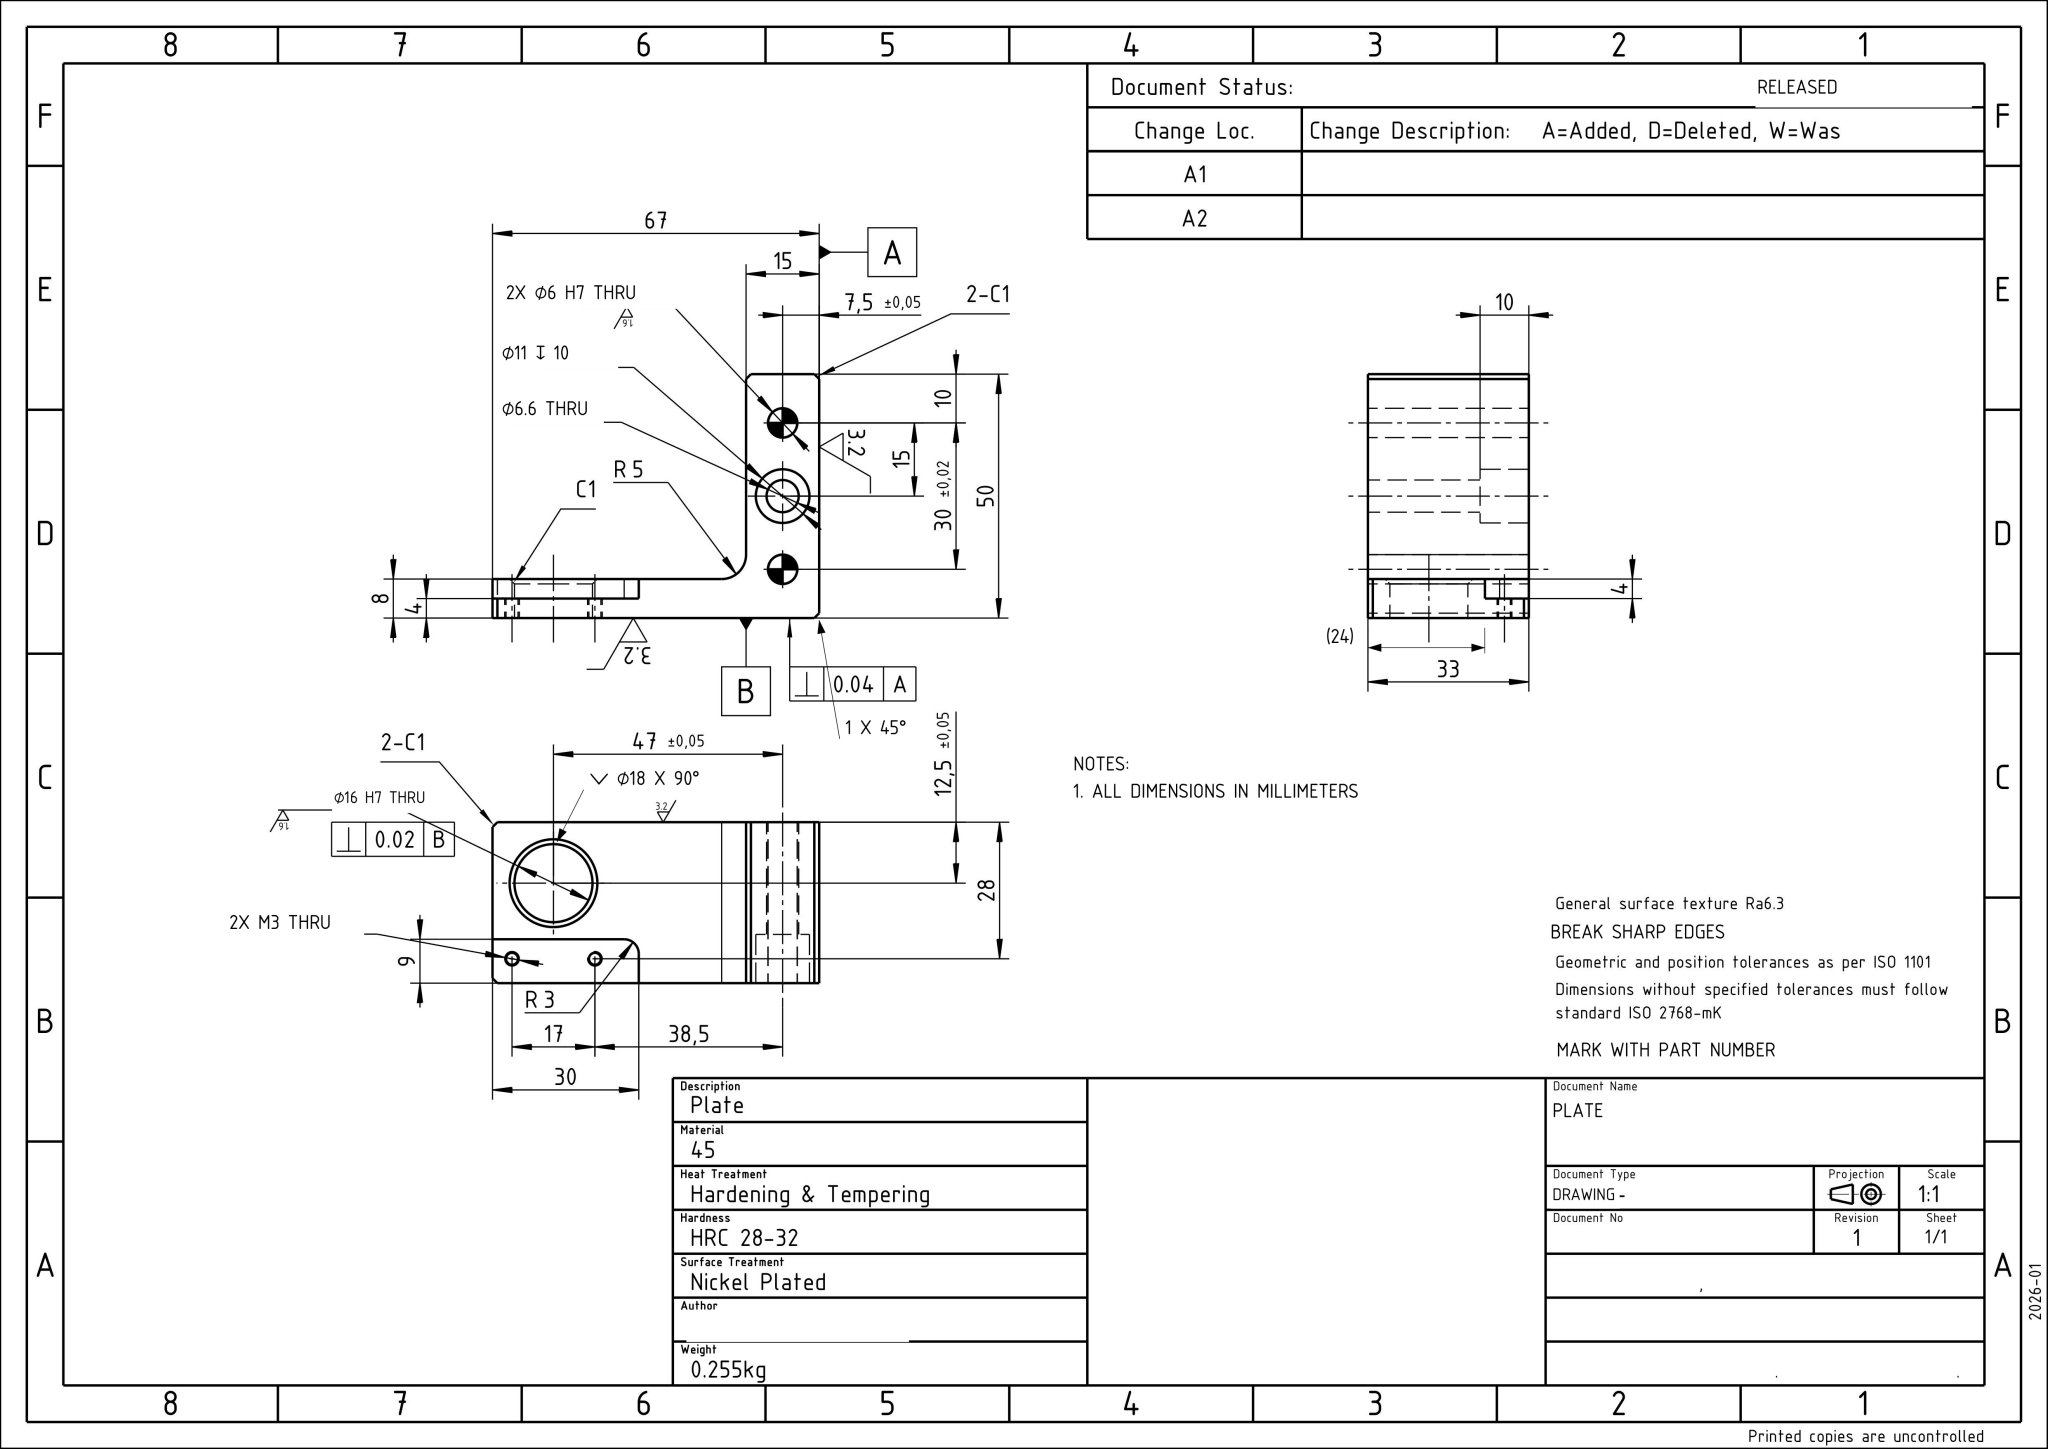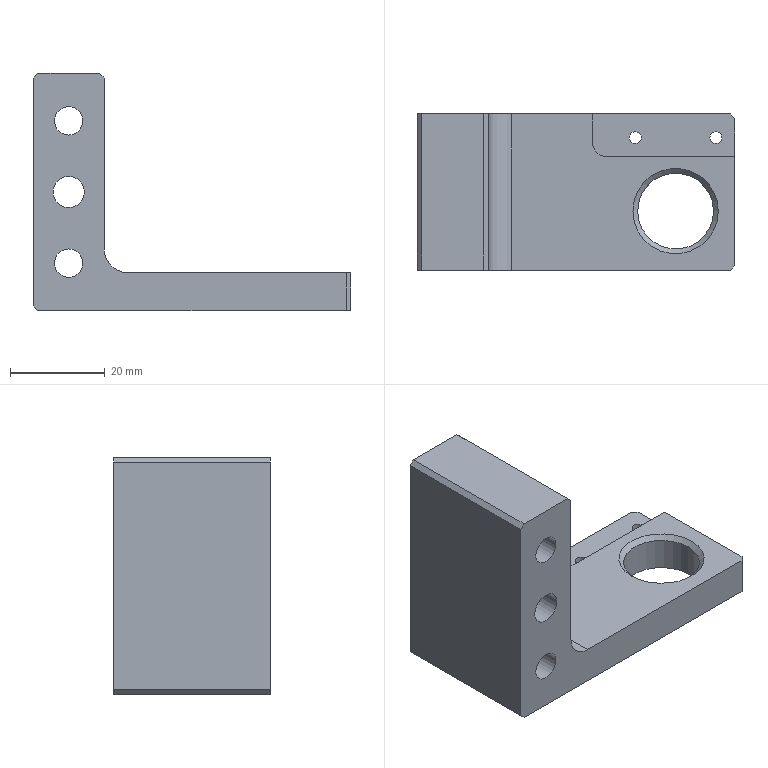Part | NX | mm | 1 solid | 27 faces | box 67 x 33 x 50 mm | volume 32250 mm3 | plane 17 | cylinder 9 | cone 1 | commonest cylinder face diameters 6 x3 2.5 x2 10 x1 16 x1 6.6 x1 11 x1
STEP:
#1=CARTESIAN_POINT('',(0.,0.,0.));
#2=DIRECTION('',(0.,0.,1.));
#3=DIRECTION('',(1.,0.,0.));
#4=AXIS2_PLACEMENT_3D('',#1,#2,#3);
#5=(LENGTH_UNIT()NAMED_UNIT(*)SI_UNIT(.MILLI.,.METRE.));
#6=UNCERTAINTY_MEASURE_WITH_UNIT(LENGTH_MEASURE(0.00002),#5,'','');
#7=(NAMED_UNIT(*)PLANE_ANGLE_UNIT()SI_UNIT($,.RADIAN.));
#8=PLANE_ANGLE_MEASURE_WITH_UNIT(PLANE_ANGLE_MEASURE(0.01745),#7);
#9=DIMENSIONAL_EXPONENTS(0.,0.,0.,0.,0.,0.,0.);
#10=(CONVERSION_BASED_UNIT('',#8)NAMED_UNIT(#9)PLANE_ANGLE_UNIT());
#11=(NAMED_UNIT(*)SI_UNIT($,.STERADIAN.)SOLID_ANGLE_UNIT());
#12=(GEOMETRIC_REPRESENTATION_CONTEXT(3)GLOBAL_UNCERTAINTY_ASSIGNED_CONTEXT((#6))GLOBAL_UNIT_ASSIGNED_CONTEXT((#5,#10,#11))REPRESENTATION_CONTEXT('',''));
#13=SHAPE_REPRESENTATION('',(#4),#12);
#14=CARTESIAN_POINT('',(45.5,-4.,8.));
#15=VERTEX_POINT('',#14);
#16=CARTESIAN_POINT('',(54.5,-4.,8.));
#17=DIRECTION('',(-0.,0.,-1.));
#18=DIRECTION('',(-1.,0.,0.));
#19=AXIS2_PLACEMENT_3D('',#16,#17,#18);
#20=CIRCLE('',#19,9.);
#21=EDGE_CURVE('',#15,#15,#20,.T.);
#22=ORIENTED_EDGE('',*,*,#21,.T.);
#23=EDGE_LOOP('',(#22));
#24=FACE_BOUND('',#23,.T.);
#25=CARTESIAN_POINT('',(66.,-16.5,8.));
#26=VERTEX_POINT('',#25);
#27=CARTESIAN_POINT('',(20.,-16.5,8.));
#28=VERTEX_POINT('',#27);
#29=CARTESIAN_POINT('',(67.,-16.5,8.));
#30=DIRECTION('',(-1.,0.,0.));
#31=VECTOR('',#30,1.);
#32=LINE('',#29,#31);
#33=EDGE_CURVE('',#26,#28,#32,.T.);
#34=ORIENTED_EDGE('',*,*,#33,.F.);
#35=CARTESIAN_POINT('',(67.,-15.5,8.));
#36=VERTEX_POINT('',#35);
#37=CARTESIAN_POINT('',(66.,-16.5,8.));
#38=DIRECTION('',(0.7071,0.7071,-0.));
#39=VECTOR('',#38,1.);
#40=LINE('',#37,#39);
#41=EDGE_CURVE('',#26,#36,#40,.T.);
#42=ORIENTED_EDGE('',*,*,#41,.T.);
#43=CARTESIAN_POINT('',(67.,7.5,8.));
#44=VERTEX_POINT('',#43);
#45=CARTESIAN_POINT('',(67.,-16.5,8.));
#46=DIRECTION('',(0.,1.,0.));
#47=VECTOR('',#46,1.);
#48=LINE('',#45,#47);
#49=EDGE_CURVE('',#36,#44,#48,.T.);
#50=ORIENTED_EDGE('',*,*,#49,.T.);
#51=CARTESIAN_POINT('',(40.,7.5,8.));
#52=VERTEX_POINT('',#51);
#53=CARTESIAN_POINT('',(37.,7.5,8.));
#54=DIRECTION('',(1.,0.,-0.));
#55=VECTOR('',#54,1.);
#56=LINE('',#53,#55);
#57=EDGE_CURVE('',#52,#44,#56,.T.);
#58=ORIENTED_EDGE('',*,*,#57,.F.);
#59=CARTESIAN_POINT('',(37.,10.5,8.));
#60=VERTEX_POINT('',#59);
#61=CARTESIAN_POINT('',(40.,10.5,8.));
#62=DIRECTION('',(-0.,0.,-1.));
#63=DIRECTION('',(-1.,0.,0.));
#64=AXIS2_PLACEMENT_3D('',#61,#62,#63);
#65=CIRCLE('',#64,3.);
#66=EDGE_CURVE('',#52,#60,#65,.T.);
#67=ORIENTED_EDGE('',*,*,#66,.T.);
#68=CARTESIAN_POINT('',(37.,16.5,8.));
#69=VERTEX_POINT('',#68);
#70=CARTESIAN_POINT('',(37.,16.5,8.));
#71=DIRECTION('',(0.,-1.,0.));
#72=VECTOR('',#71,1.);
#73=LINE('',#70,#72);
#74=EDGE_CURVE('',#69,#60,#73,.T.);
#75=ORIENTED_EDGE('',*,*,#74,.F.);
#76=CARTESIAN_POINT('',(20.,16.5,8.));
#77=VERTEX_POINT('',#76);
#78=CARTESIAN_POINT('',(67.,16.5,8.));
#79=DIRECTION('',(-1.,0.,0.));
#80=VECTOR('',#79,1.);
#81=LINE('',#78,#80);
#82=EDGE_CURVE('',#69,#77,#81,.T.);
#83=ORIENTED_EDGE('',*,*,#82,.T.);
#84=CARTESIAN_POINT('',(20.,-16.5,8.));
#85=DIRECTION('',(0.,-1.,0.));
#86=VECTOR('',#85,1.);
#87=LINE('',#84,#86);
#88=EDGE_CURVE('',#77,#28,#87,.T.);
#89=ORIENTED_EDGE('',*,*,#88,.T.);
#90=EDGE_LOOP('',(#34,#42,#50,#58,#67,#75,#83,#89));
#91=FACE_BOUND('',#90,.T.);
#92=CARTESIAN_POINT('',(67.,-16.5,8.));
#93=DIRECTION('',(-0.,0.,-1.));
#94=DIRECTION('',(-1.,0.,0.));
#95=AXIS2_PLACEMENT_3D('',#92,#93,#94);
#96=PLANE('',#95);
#97=ADVANCED_FACE('',(#24,#91),#96,.F.);
#98=CARTESIAN_POINT('',(7.5,16.5,37.));
#99=VERTEX_POINT('',#98);
#100=CARTESIAN_POINT('',(7.5,16.5,40.));
#101=DIRECTION('',(0.,-1.,0.));
#102=DIRECTION('',(0.,0.,-1.));
#103=AXIS2_PLACEMENT_3D('',#100,#101,#102);
#104=CIRCLE('',#103,3.);
#105=EDGE_CURVE('',#99,#99,#104,.T.);
#106=ORIENTED_EDGE('',*,*,#105,.T.);
#107=EDGE_LOOP('',(#106));
#108=FACE_BOUND('',#107,.T.);
#109=CARTESIAN_POINT('',(7.5,16.5,7.));
#110=VERTEX_POINT('',#109);
#111=CARTESIAN_POINT('',(7.5,16.5,10.));
#112=DIRECTION('',(0.,-1.,0.));
#113=DIRECTION('',(0.,0.,-1.));
#114=AXIS2_PLACEMENT_3D('',#111,#112,#113);
#115=CIRCLE('',#114,3.);
#116=EDGE_CURVE('',#110,#110,#115,.T.);
#117=ORIENTED_EDGE('',*,*,#116,.T.);
#118=EDGE_LOOP('',(#117));
#119=FACE_BOUND('',#118,.T.);
#120=CARTESIAN_POINT('',(7.5,16.5,19.5));
#121=VERTEX_POINT('',#120);
#122=CARTESIAN_POINT('',(7.5,16.5,25.));
#123=DIRECTION('',(0.,-1.,0.));
#124=DIRECTION('',(0.,0.,-1.));
#125=AXIS2_PLACEMENT_3D('',#122,#123,#124);
#126=CIRCLE('',#125,5.5);
#127=EDGE_CURVE('',#121,#121,#126,.T.);
#128=ORIENTED_EDGE('',*,*,#127,.T.);
#129=EDGE_LOOP('',(#128));
#130=FACE_BOUND('',#129,.T.);
#131=CARTESIAN_POINT('',(66.,16.5,4.));
#132=VERTEX_POINT('',#131);
#133=CARTESIAN_POINT('',(37.,16.5,4.));
#134=VERTEX_POINT('',#133);
#135=CARTESIAN_POINT('',(67.,16.5,4.));
#136=DIRECTION('',(-1.,0.,0.));
#137=VECTOR('',#136,1.);
#138=LINE('',#135,#137);
#139=EDGE_CURVE('',#132,#134,#138,.T.);
#140=ORIENTED_EDGE('',*,*,#139,.F.);
#141=CARTESIAN_POINT('',(66.,16.5,0.));
#142=VERTEX_POINT('',#141);
#143=CARTESIAN_POINT('',(66.,16.5,-0.));
#144=DIRECTION('',(-0.,0.,-1.));
#145=VECTOR('',#144,1.);
#146=LINE('',#143,#145);
#147=EDGE_CURVE('',#132,#142,#146,.T.);
#148=ORIENTED_EDGE('',*,*,#147,.T.);
#149=CARTESIAN_POINT('',(1.,16.5,0.));
#150=VERTEX_POINT('',#149);
#151=CARTESIAN_POINT('',(-0.,16.5,0.));
#152=DIRECTION('',(1.,0.,0.));
#153=VECTOR('',#152,1.);
#154=LINE('',#151,#153);
#155=EDGE_CURVE('',#150,#142,#154,.T.);
#156=ORIENTED_EDGE('',*,*,#155,.F.);
#157=CARTESIAN_POINT('',(-0.,16.5,1.));
#158=VERTEX_POINT('',#157);
#159=CARTESIAN_POINT('',(1.,16.5,0.));
#160=DIRECTION('',(-0.7071,0.,0.7071));
#161=VECTOR('',#160,1.);
#162=LINE('',#159,#161);
#163=EDGE_CURVE('',#150,#158,#162,.T.);
#164=ORIENTED_EDGE('',*,*,#163,.T.);
#165=CARTESIAN_POINT('',(0.,16.5,49.));
#166=VERTEX_POINT('',#165);
#167=CARTESIAN_POINT('',(0.,16.5,50.));
#168=DIRECTION('',(-0.,0.,-1.));
#169=VECTOR('',#168,1.);
#170=LINE('',#167,#169);
#171=EDGE_CURVE('',#166,#158,#170,.T.);
#172=ORIENTED_EDGE('',*,*,#171,.F.);
#173=CARTESIAN_POINT('',(1.,16.5,50.));
#174=VERTEX_POINT('',#173);
#175=CARTESIAN_POINT('',(0.,16.5,49.));
#176=DIRECTION('',(0.7071,0.,0.7071));
#177=VECTOR('',#176,1.);
#178=LINE('',#175,#177);
#179=EDGE_CURVE('',#166,#174,#178,.T.);
#180=ORIENTED_EDGE('',*,*,#179,.T.);
#181=CARTESIAN_POINT('',(14.,16.5,50.));
#182=VERTEX_POINT('',#181);
#183=CARTESIAN_POINT('',(15.,16.5,50.));
#184=DIRECTION('',(-1.,0.,0.));
#185=VECTOR('',#184,1.);
#186=LINE('',#183,#185);
#187=EDGE_CURVE('',#182,#174,#186,.T.);
#188=ORIENTED_EDGE('',*,*,#187,.F.);
#189=CARTESIAN_POINT('',(15.,16.5,49.));
#190=VERTEX_POINT('',#189);
#191=CARTESIAN_POINT('',(14.,16.5,50.));
#192=DIRECTION('',(0.7071,0.,-0.7071));
#193=VECTOR('',#192,1.);
#194=LINE('',#191,#193);
#195=EDGE_CURVE('',#182,#190,#194,.T.);
#196=ORIENTED_EDGE('',*,*,#195,.T.);
#197=CARTESIAN_POINT('',(15.,16.5,13.));
#198=VERTEX_POINT('',#197);
#199=CARTESIAN_POINT('',(15.,16.5,8.));
#200=DIRECTION('',(0.,0.,1.));
#201=VECTOR('',#200,1.);
#202=LINE('',#199,#201);
#203=EDGE_CURVE('',#198,#190,#202,.T.);
#204=ORIENTED_EDGE('',*,*,#203,.F.);
#205=CARTESIAN_POINT('',(20.,16.5,13.));
#206=DIRECTION('',(0.,-1.,0.));
#207=DIRECTION('',(0.,0.,-1.));
#208=AXIS2_PLACEMENT_3D('',#205,#206,#207);
#209=CIRCLE('',#208,5.);
#210=EDGE_CURVE('',#198,#77,#209,.T.);
#211=ORIENTED_EDGE('',*,*,#210,.T.);
#212=ORIENTED_EDGE('',*,*,#82,.F.);
#213=CARTESIAN_POINT('',(37.,16.5,4.));
#214=DIRECTION('',(0.,0.,1.));
#215=VECTOR('',#214,1.);
#216=LINE('',#213,#215);
#217=EDGE_CURVE('',#134,#69,#216,.T.);
#218=ORIENTED_EDGE('',*,*,#217,.F.);
#219=EDGE_LOOP('',(#140,#148,#156,#164,#172,#180,#188,#196,#204,#211,#212,#218));
#220=FACE_BOUND('',#219,.T.);
#221=CARTESIAN_POINT('',(0.,16.5,0.));
#222=DIRECTION('',(0.,-1.,0.));
#223=DIRECTION('',(0.,0.,-1.));
#224=AXIS2_PLACEMENT_3D('',#221,#222,#223);
#225=PLANE('',#224);
#226=ADVANCED_FACE('',(#108,#119,#130,#220),#225,.F.);
#227=CARTESIAN_POINT('',(0.,-16.5,49.));
#228=VERTEX_POINT('',#227);
#229=CARTESIAN_POINT('',(-0.,-16.5,1.));
#230=VERTEX_POINT('',#229);
#231=CARTESIAN_POINT('',(0.,-16.5,50.));
#232=DIRECTION('',(-0.,0.,-1.));
#233=VECTOR('',#232,1.);
#234=LINE('',#231,#233);
#235=EDGE_CURVE('',#228,#230,#234,.T.);
#236=ORIENTED_EDGE('',*,*,#235,.F.);
#237=CARTESIAN_POINT('',(0.,-16.5,49.));
#238=DIRECTION('',(0.,1.,0.));
#239=VECTOR('',#238,1.);
#240=LINE('',#237,#239);
#241=EDGE_CURVE('',#228,#166,#240,.T.);
#242=ORIENTED_EDGE('',*,*,#241,.T.);
#243=ORIENTED_EDGE('',*,*,#171,.T.);
#244=CARTESIAN_POINT('',(-0.,-16.5,1.));
#245=DIRECTION('',(0.,-1.,0.));
#246=VECTOR('',#245,1.);
#247=LINE('',#244,#246);
#248=EDGE_CURVE('',#158,#230,#247,.T.);
#249=ORIENTED_EDGE('',*,*,#248,.T.);
#250=EDGE_LOOP('',(#236,#242,#243,#249));
#251=FACE_OUTER_BOUND('',#250,.T.);
#252=CARTESIAN_POINT('',(0.,-16.5,50.));
#253=DIRECTION('',(1.,0.,-0.));
#254=DIRECTION('',(-0.,0.,-1.));
#255=AXIS2_PLACEMENT_3D('',#252,#253,#254);
#256=PLANE('',#255);
#257=ADVANCED_FACE('',(#251),#256,.F.);
#258=CARTESIAN_POINT('',(64.25,11.5,0.));
#259=VERTEX_POINT('',#258);
#260=CARTESIAN_POINT('',(63.,11.5,0.));
#261=DIRECTION('',(0.,0.,1.));
#262=DIRECTION('',(1.,0.,0.));
#263=AXIS2_PLACEMENT_3D('',#260,#261,#262);
#264=CIRCLE('',#263,1.25);
#265=EDGE_CURVE('',#259,#259,#264,.T.);
#266=ORIENTED_EDGE('',*,*,#265,.T.);
#267=EDGE_LOOP('',(#266));
#268=FACE_BOUND('',#267,.T.);
#269=CARTESIAN_POINT('',(47.25,11.5,0.));
#270=VERTEX_POINT('',#269);
#271=CARTESIAN_POINT('',(46.,11.5,0.));
#272=DIRECTION('',(0.,0.,1.));
#273=DIRECTION('',(1.,0.,0.));
#274=AXIS2_PLACEMENT_3D('',#271,#272,#273);
#275=CIRCLE('',#274,1.25);
#276=EDGE_CURVE('',#270,#270,#275,.T.);
#277=ORIENTED_EDGE('',*,*,#276,.T.);
#278=EDGE_LOOP('',(#277));
#279=FACE_BOUND('',#278,.T.);
#280=CARTESIAN_POINT('',(62.5,-4.,0.));
#281=VERTEX_POINT('',#280);
#282=CARTESIAN_POINT('',(54.5,-4.,0.));
#283=DIRECTION('',(0.,0.,1.));
#284=DIRECTION('',(1.,0.,0.));
#285=AXIS2_PLACEMENT_3D('',#282,#283,#284);
#286=CIRCLE('',#285,8.);
#287=EDGE_CURVE('',#281,#281,#286,.T.);
#288=ORIENTED_EDGE('',*,*,#287,.T.);
#289=EDGE_LOOP('',(#288));
#290=FACE_BOUND('',#289,.T.);
#291=ORIENTED_EDGE('',*,*,#155,.T.);
#292=CARTESIAN_POINT('',(67.,15.5,0.));
#293=VERTEX_POINT('',#292);
#294=CARTESIAN_POINT('',(67.,15.5,0.));
#295=DIRECTION('',(0.7071,-0.7071,0.));
#296=VECTOR('',#295,1.);
#297=LINE('',#294,#296);
#298=EDGE_CURVE('',#142,#293,#297,.T.);
#299=ORIENTED_EDGE('',*,*,#298,.T.);
#300=CARTESIAN_POINT('',(67.,-15.5,0.));
#301=VERTEX_POINT('',#300);
#302=CARTESIAN_POINT('',(67.,-16.5,0.));
#303=DIRECTION('',(0.,1.,0.));
#304=VECTOR('',#303,1.);
#305=LINE('',#302,#304);
#306=EDGE_CURVE('',#301,#293,#305,.T.);
#307=ORIENTED_EDGE('',*,*,#306,.F.);
#308=CARTESIAN_POINT('',(66.,-16.5,0.));
#309=VERTEX_POINT('',#308);
#310=CARTESIAN_POINT('',(66.,-16.5,0.));
#311=DIRECTION('',(-0.7071,-0.7071,0.));
#312=VECTOR('',#311,1.);
#313=LINE('',#310,#312);
#314=EDGE_CURVE('',#301,#309,#313,.T.);
#315=ORIENTED_EDGE('',*,*,#314,.T.);
#316=CARTESIAN_POINT('',(1.,-16.5,0.));
#317=VERTEX_POINT('',#316);
#318=CARTESIAN_POINT('',(-0.,-16.5,0.));
#319=DIRECTION('',(1.,0.,0.));
#320=VECTOR('',#319,1.);
#321=LINE('',#318,#320);
#322=EDGE_CURVE('',#317,#309,#321,.T.);
#323=ORIENTED_EDGE('',*,*,#322,.F.);
#324=CARTESIAN_POINT('',(1.,-16.5,0.));
#325=DIRECTION('',(0.,1.,0.));
#326=VECTOR('',#325,1.);
#327=LINE('',#324,#326);
#328=EDGE_CURVE('',#317,#150,#327,.T.);
#329=ORIENTED_EDGE('',*,*,#328,.T.);
#330=EDGE_LOOP('',(#291,#299,#307,#315,#323,#329));
#331=FACE_BOUND('',#330,.T.);
#332=CARTESIAN_POINT('',(-0.,-16.5,0.));
#333=DIRECTION('',(0.,0.,1.));
#334=DIRECTION('',(1.,0.,0.));
#335=AXIS2_PLACEMENT_3D('',#332,#333,#334);
#336=PLANE('',#335);
#337=ADVANCED_FACE('',(#268,#279,#290,#331),#336,.F.);
#338=ORIENTED_EDGE('',*,*,#306,.T.);
#339=CARTESIAN_POINT('',(67.,15.5,4.));
#340=VERTEX_POINT('',#339);
#341=CARTESIAN_POINT('',(67.,15.5,0.));
#342=DIRECTION('',(0.,0.,1.));
#343=VECTOR('',#342,1.);
#344=LINE('',#341,#343);
#345=EDGE_CURVE('',#293,#340,#344,.T.);
#346=ORIENTED_EDGE('',*,*,#345,.T.);
#347=CARTESIAN_POINT('',(67.,7.5,4.));
#348=VERTEX_POINT('',#347);
#349=CARTESIAN_POINT('',(67.,7.5,4.));
#350=DIRECTION('',(0.,1.,0.));
#351=VECTOR('',#350,1.);
#352=LINE('',#349,#351);
#353=EDGE_CURVE('',#348,#340,#352,.T.);
#354=ORIENTED_EDGE('',*,*,#353,.F.);
#355=CARTESIAN_POINT('',(67.,7.5,4.));
#356=DIRECTION('',(0.,0.,1.));
#357=VECTOR('',#356,1.);
#358=LINE('',#355,#357);
#359=EDGE_CURVE('',#348,#44,#358,.T.);
#360=ORIENTED_EDGE('',*,*,#359,.T.);
#361=ORIENTED_EDGE('',*,*,#49,.F.);
#362=CARTESIAN_POINT('',(67.,-15.5,-0.));
#363=DIRECTION('',(-0.,0.,-1.));
#364=VECTOR('',#363,1.);
#365=LINE('',#362,#364);
#366=EDGE_CURVE('',#36,#301,#365,.T.);
#367=ORIENTED_EDGE('',*,*,#366,.T.);
#368=EDGE_LOOP('',(#338,#346,#354,#360,#361,#367));
#369=FACE_OUTER_BOUND('',#368,.T.);
#370=CARTESIAN_POINT('',(67.,-16.5,0.));
#371=DIRECTION('',(-1.,0.,0.));
#372=DIRECTION('',(0.,0.,1.));
#373=AXIS2_PLACEMENT_3D('',#370,#371,#372);
#374=PLANE('',#373);
#375=ADVANCED_FACE('',(#369),#374,.F.);
#376=ORIENTED_EDGE('',*,*,#203,.T.);
#377=CARTESIAN_POINT('',(15.,-16.5,49.));
#378=VERTEX_POINT('',#377);
#379=CARTESIAN_POINT('',(15.,-16.5,49.));
#380=DIRECTION('',(0.,-1.,0.));
#381=VECTOR('',#380,1.);
#382=LINE('',#379,#381);
#383=EDGE_CURVE('',#190,#378,#382,.T.);
#384=ORIENTED_EDGE('',*,*,#383,.T.);
#385=CARTESIAN_POINT('',(15.,-16.5,13.));
#386=VERTEX_POINT('',#385);
#387=CARTESIAN_POINT('',(15.,-16.5,8.));
#388=DIRECTION('',(0.,0.,1.));
#389=VECTOR('',#388,1.);
#390=LINE('',#387,#389);
#391=EDGE_CURVE('',#386,#378,#390,.T.);
#392=ORIENTED_EDGE('',*,*,#391,.F.);
#393=CARTESIAN_POINT('',(15.,16.5,13.));
#394=DIRECTION('',(0.,1.,0.));
#395=VECTOR('',#394,1.);
#396=LINE('',#393,#395);
#397=EDGE_CURVE('',#386,#198,#396,.T.);
#398=ORIENTED_EDGE('',*,*,#397,.T.);
#399=EDGE_LOOP('',(#376,#384,#392,#398));
#400=FACE_OUTER_BOUND('',#399,.T.);
#401=CARTESIAN_POINT('',(15.,-16.5,8.));
#402=DIRECTION('',(-1.,0.,0.));
#403=DIRECTION('',(0.,0.,1.));
#404=AXIS2_PLACEMENT_3D('',#401,#402,#403);
#405=PLANE('',#404);
#406=ADVANCED_FACE('',(#400),#405,.F.);
#407=ORIENTED_EDGE('',*,*,#187,.T.);
#408=CARTESIAN_POINT('',(1.,-16.5,50.));
#409=VERTEX_POINT('',#408);
#410=CARTESIAN_POINT('',(1.,-16.5,50.));
#411=DIRECTION('',(0.,-1.,0.));
#412=VECTOR('',#411,1.);
#413=LINE('',#410,#412);
#414=EDGE_CURVE('',#174,#409,#413,.T.);
#415=ORIENTED_EDGE('',*,*,#414,.T.);
#416=CARTESIAN_POINT('',(14.,-16.5,50.));
#417=VERTEX_POINT('',#416);
#418=CARTESIAN_POINT('',(15.,-16.5,50.));
#419=DIRECTION('',(-1.,0.,0.));
#420=VECTOR('',#419,1.);
#421=LINE('',#418,#420);
#422=EDGE_CURVE('',#417,#409,#421,.T.);
#423=ORIENTED_EDGE('',*,*,#422,.F.);
#424=CARTESIAN_POINT('',(14.,-16.5,50.));
#425=DIRECTION('',(0.,1.,0.));
#426=VECTOR('',#425,1.);
#427=LINE('',#424,#426);
#428=EDGE_CURVE('',#417,#182,#427,.T.);
#429=ORIENTED_EDGE('',*,*,#428,.T.);
#430=EDGE_LOOP('',(#407,#415,#423,#429));
#431=FACE_OUTER_BOUND('',#430,.T.);
#432=CARTESIAN_POINT('',(15.,-16.5,50.));
#433=DIRECTION('',(-0.,0.,-1.));
#434=DIRECTION('',(-1.,0.,0.));
#435=AXIS2_PLACEMENT_3D('',#432,#433,#434);
#436=PLANE('',#435);
#437=ADVANCED_FACE('',(#431),#436,.F.);
#438=CARTESIAN_POINT('',(7.5,-16.5,37.));
#439=VERTEX_POINT('',#438);
#440=CARTESIAN_POINT('',(7.5,-16.5,40.));
#441=DIRECTION('',(0.,-1.,0.));
#442=DIRECTION('',(0.,0.,-1.));
#443=AXIS2_PLACEMENT_3D('',#440,#441,#442);
#444=CIRCLE('',#443,3.);
#445=EDGE_CURVE('',#439,#439,#444,.T.);
#446=ORIENTED_EDGE('',*,*,#445,.F.);
#447=EDGE_LOOP('',(#446));
#448=FACE_BOUND('',#447,.T.);
#449=CARTESIAN_POINT('',(7.5,-16.5,7.));
#450=VERTEX_POINT('',#449);
#451=CARTESIAN_POINT('',(7.5,-16.5,10.));
#452=DIRECTION('',(0.,-1.,0.));
#453=DIRECTION('',(0.,0.,-1.));
#454=AXIS2_PLACEMENT_3D('',#451,#452,#453);
#455=CIRCLE('',#454,3.);
#456=EDGE_CURVE('',#450,#450,#455,.T.);
#457=ORIENTED_EDGE('',*,*,#456,.F.);
#458=EDGE_LOOP('',(#457));
#459=FACE_BOUND('',#458,.T.);
#460=CARTESIAN_POINT('',(7.5,-16.5,21.7));
#461=VERTEX_POINT('',#460);
#462=CARTESIAN_POINT('',(7.5,-16.5,25.));
#463=DIRECTION('',(0.,-1.,0.));
#464=DIRECTION('',(0.,0.,-1.));
#465=AXIS2_PLACEMENT_3D('',#462,#463,#464);
#466=CIRCLE('',#465,3.3);
#467=EDGE_CURVE('',#461,#461,#466,.T.);
#468=ORIENTED_EDGE('',*,*,#467,.F.);
#469=EDGE_LOOP('',(#468));
#470=FACE_BOUND('',#469,.T.);
#471=ORIENTED_EDGE('',*,*,#322,.T.);
#472=CARTESIAN_POINT('',(66.,-16.5,8.));
#473=DIRECTION('',(0.,0.,1.));
#474=VECTOR('',#473,1.);
#475=LINE('',#472,#474);
#476=EDGE_CURVE('',#309,#26,#475,.T.);
#477=ORIENTED_EDGE('',*,*,#476,.T.);
#478=ORIENTED_EDGE('',*,*,#33,.T.);
#479=CARTESIAN_POINT('',(20.,-16.5,13.));
#480=DIRECTION('',(0.,1.,0.));
#481=DIRECTION('',(0.,0.,-1.));
#482=AXIS2_PLACEMENT_3D('',#479,#480,#481);
#483=CIRCLE('',#482,5.);
#484=EDGE_CURVE('',#28,#386,#483,.T.);
#485=ORIENTED_EDGE('',*,*,#484,.T.);
#486=ORIENTED_EDGE('',*,*,#391,.T.);
#487=CARTESIAN_POINT('',(32.,-16.5,32.));
#488=DIRECTION('',(-0.7071,0.,0.7071));
#489=VECTOR('',#488,1.);
#490=LINE('',#487,#489);
#491=EDGE_CURVE('',#378,#417,#490,.T.);
#492=ORIENTED_EDGE('',*,*,#491,.T.);
#493=ORIENTED_EDGE('',*,*,#422,.T.);
#494=CARTESIAN_POINT('',(-24.5,-16.5,24.5));
#495=DIRECTION('',(-0.7071,0.,-0.7071));
#496=VECTOR('',#495,1.);
#497=LINE('',#494,#496);
#498=EDGE_CURVE('',#409,#228,#497,.T.);
#499=ORIENTED_EDGE('',*,*,#498,.T.);
#500=ORIENTED_EDGE('',*,*,#235,.T.);
#501=CARTESIAN_POINT('',(0.5,-16.5,0.5));
#502=DIRECTION('',(0.7071,0.,-0.7071));
#503=VECTOR('',#502,1.);
#504=LINE('',#501,#503);
#505=EDGE_CURVE('',#230,#317,#504,.T.);
#506=ORIENTED_EDGE('',*,*,#505,.T.);
#507=EDGE_LOOP('',(#471,#477,#478,#485,#486,#492,#493,#499,#500,#506));
#508=FACE_BOUND('',#507,.T.);
#509=CARTESIAN_POINT('',(0.,-16.5,0.));
#510=DIRECTION('',(0.,-1.,0.));
#511=DIRECTION('',(0.,0.,-1.));
#512=AXIS2_PLACEMENT_3D('',#509,#510,#511);
#513=PLANE('',#512);
#514=ADVANCED_FACE('',(#448,#459,#470,#508),#513,.T.);
#515=ORIENTED_EDGE('',*,*,#74,.T.);
#516=CARTESIAN_POINT('',(37.,10.5,4.));
#517=VERTEX_POINT('',#516);
#518=CARTESIAN_POINT('',(37.,10.5,4.));
#519=DIRECTION('',(-0.,0.,-1.));
#520=VECTOR('',#519,1.);
#521=LINE('',#518,#520);
#522=EDGE_CURVE('',#60,#517,#521,.T.);
#523=ORIENTED_EDGE('',*,*,#522,.T.);
#524=CARTESIAN_POINT('',(37.,16.5,4.));
#525=DIRECTION('',(0.,1.,0.));
#526=VECTOR('',#525,1.);
#527=LINE('',#524,#526);
#528=EDGE_CURVE('',#517,#134,#527,.T.);
#529=ORIENTED_EDGE('',*,*,#528,.T.);
#530=ORIENTED_EDGE('',*,*,#217,.T.);
#531=EDGE_LOOP('',(#515,#523,#529,#530));
#532=FACE_OUTER_BOUND('',#531,.T.);
#533=CARTESIAN_POINT('',(37.,16.5,4.));
#534=DIRECTION('',(-1.,0.,0.));
#535=DIRECTION('',(0.,0.,1.));
#536=AXIS2_PLACEMENT_3D('',#533,#534,#535);
#537=PLANE('',#536);
#538=ADVANCED_FACE('',(#532),#537,.F.);
#539=CARTESIAN_POINT('',(40.,7.5,4.));
#540=VERTEX_POINT('',#539);
#541=CARTESIAN_POINT('',(37.,7.5,4.));
#542=DIRECTION('',(-1.,0.,0.));
#543=VECTOR('',#542,1.);
#544=LINE('',#541,#543);
#545=EDGE_CURVE('',#348,#540,#544,.T.);
#546=ORIENTED_EDGE('',*,*,#545,.T.);
#547=CARTESIAN_POINT('',(40.,7.5,8.));
#548=DIRECTION('',(0.,0.,1.));
#549=VECTOR('',#548,1.);
#550=LINE('',#547,#549);
#551=EDGE_CURVE('',#540,#52,#550,.T.);
#552=ORIENTED_EDGE('',*,*,#551,.T.);
#553=ORIENTED_EDGE('',*,*,#57,.T.);
#554=ORIENTED_EDGE('',*,*,#359,.F.);
#555=EDGE_LOOP('',(#546,#552,#553,#554));
#556=FACE_OUTER_BOUND('',#555,.T.);
#557=CARTESIAN_POINT('',(37.,7.5,4.));
#558=DIRECTION('',(0.,-1.,0.));
#559=DIRECTION('',(0.,0.,-1.));
#560=AXIS2_PLACEMENT_3D('',#557,#558,#559);
#561=PLANE('',#560);
#562=ADVANCED_FACE('',(#556),#561,.F.);
#563=CARTESIAN_POINT('',(61.75,11.5,4.));
#564=VERTEX_POINT('',#563);
#565=CARTESIAN_POINT('',(63.,11.5,4.));
#566=DIRECTION('',(-0.,0.,-1.));
#567=DIRECTION('',(-1.,0.,0.));
#568=AXIS2_PLACEMENT_3D('',#565,#566,#567);
#569=CIRCLE('',#568,1.25);
#570=EDGE_CURVE('',#564,#564,#569,.T.);
#571=ORIENTED_EDGE('',*,*,#570,.T.);
#572=EDGE_LOOP('',(#571));
#573=FACE_BOUND('',#572,.T.);
#574=CARTESIAN_POINT('',(44.75,11.5,4.));
#575=VERTEX_POINT('',#574);
#576=CARTESIAN_POINT('',(46.,11.5,4.));
#577=DIRECTION('',(-0.,0.,-1.));
#578=DIRECTION('',(-1.,0.,0.));
#579=AXIS2_PLACEMENT_3D('',#576,#577,#578);
#580=CIRCLE('',#579,1.25);
#581=EDGE_CURVE('',#575,#575,#580,.T.);
#582=ORIENTED_EDGE('',*,*,#581,.T.);
#583=EDGE_LOOP('',(#582));
#584=FACE_BOUND('',#583,.T.);
#585=ORIENTED_EDGE('',*,*,#353,.T.);
#586=CARTESIAN_POINT('',(41.25,41.25,4.));
#587=DIRECTION('',(-0.7071,0.7071,0.));
#588=VECTOR('',#587,1.);
#589=LINE('',#586,#588);
#590=EDGE_CURVE('',#340,#132,#589,.T.);
#591=ORIENTED_EDGE('',*,*,#590,.T.);
#592=ORIENTED_EDGE('',*,*,#139,.T.);
#593=ORIENTED_EDGE('',*,*,#528,.F.);
#594=CARTESIAN_POINT('',(40.,10.5,4.));
#595=DIRECTION('',(0.,0.,1.));
#596=DIRECTION('',(1.,0.,-0.));
#597=AXIS2_PLACEMENT_3D('',#594,#595,#596);
#598=CIRCLE('',#597,3.);
#599=EDGE_CURVE('',#517,#540,#598,.T.);
#600=ORIENTED_EDGE('',*,*,#599,.T.);
#601=ORIENTED_EDGE('',*,*,#545,.F.);
#602=EDGE_LOOP('',(#585,#591,#592,#593,#600,#601));
#603=FACE_BOUND('',#602,.T.);
#604=CARTESIAN_POINT('',(0.,0.,4.));
#605=DIRECTION('',(0.,0.,1.));
#606=DIRECTION('',(1.,0.,-0.));
#607=AXIS2_PLACEMENT_3D('',#604,#605,#606);
#608=PLANE('',#607);
#609=ADVANCED_FACE('',(#573,#584,#603),#608,.T.);
#610=ORIENTED_EDGE('',*,*,#66,.F.);
#611=ORIENTED_EDGE('',*,*,#551,.F.);
#612=ORIENTED_EDGE('',*,*,#599,.F.);
#613=ORIENTED_EDGE('',*,*,#522,.F.);
#614=EDGE_LOOP('',(#610,#611,#612,#613));
#615=FACE_OUTER_BOUND('',#614,.T.);
#616=CARTESIAN_POINT('',(40.,10.5,4.));
#617=DIRECTION('',(0.,0.,1.));
#618=DIRECTION('',(1.,0.,-0.));
#619=AXIS2_PLACEMENT_3D('',#616,#617,#618);
#620=CYLINDRICAL_SURFACE('',#619,3.);
#621=ADVANCED_FACE('',(#615),#620,.F.);
#622=ORIENTED_EDGE('',*,*,#484,.F.);
#623=ORIENTED_EDGE('',*,*,#88,.F.);
#624=ORIENTED_EDGE('',*,*,#210,.F.);
#625=ORIENTED_EDGE('',*,*,#397,.F.);
#626=EDGE_LOOP('',(#622,#623,#624,#625));
#627=FACE_OUTER_BOUND('',#626,.T.);
#628=CARTESIAN_POINT('',(20.,-16.5,13.));
#629=DIRECTION('',(0.,-1.,0.));
#630=DIRECTION('',(0.,0.,-1.));
#631=AXIS2_PLACEMENT_3D('',#628,#629,#630);
#632=CYLINDRICAL_SURFACE('',#631,5.);
#633=ADVANCED_FACE('',(#627),#632,.F.);
#634=ORIENTED_EDGE('',*,*,#298,.F.);
#635=ORIENTED_EDGE('',*,*,#147,.F.);
#636=ORIENTED_EDGE('',*,*,#590,.F.);
#637=ORIENTED_EDGE('',*,*,#345,.F.);
#638=EDGE_LOOP('',(#634,#635,#636,#637));
#639=FACE_OUTER_BOUND('',#638,.T.);
#640=CARTESIAN_POINT('',(67.,15.5,0.));
#641=DIRECTION('',(-0.7071,-0.7071,0.));
#642=DIRECTION('',(0.,0.,1.));
#643=AXIS2_PLACEMENT_3D('',#640,#641,#642);
#644=PLANE('',#643);
#645=ADVANCED_FACE('',(#639),#644,.F.);
#646=ORIENTED_EDGE('',*,*,#314,.F.);
#647=ORIENTED_EDGE('',*,*,#366,.F.);
#648=ORIENTED_EDGE('',*,*,#41,.F.);
#649=ORIENTED_EDGE('',*,*,#476,.F.);
#650=EDGE_LOOP('',(#646,#647,#648,#649));
#651=FACE_OUTER_BOUND('',#650,.T.);
#652=CARTESIAN_POINT('',(66.,-16.5,-0.));
#653=DIRECTION('',(0.7071,-0.7071,-0.));
#654=DIRECTION('',(-0.,0.,-1.));
#655=AXIS2_PLACEMENT_3D('',#652,#653,#654);
#656=PLANE('',#655);
#657=ADVANCED_FACE('',(#651),#656,.T.);
#658=ORIENTED_EDGE('',*,*,#498,.F.);
#659=ORIENTED_EDGE('',*,*,#414,.F.);
#660=ORIENTED_EDGE('',*,*,#179,.F.);
#661=ORIENTED_EDGE('',*,*,#241,.F.);
#662=EDGE_LOOP('',(#658,#659,#660,#661));
#663=FACE_OUTER_BOUND('',#662,.T.);
#664=CARTESIAN_POINT('',(0.,-16.5,49.));
#665=DIRECTION('',(0.7071,0.,-0.7071));
#666=DIRECTION('',(0.,1.,0.));
#667=AXIS2_PLACEMENT_3D('',#664,#665,#666);
#668=PLANE('',#667);
#669=ADVANCED_FACE('',(#663),#668,.F.);
#670=ORIENTED_EDGE('',*,*,#491,.F.);
#671=ORIENTED_EDGE('',*,*,#383,.F.);
#672=ORIENTED_EDGE('',*,*,#195,.F.);
#673=ORIENTED_EDGE('',*,*,#428,.F.);
#674=EDGE_LOOP('',(#670,#671,#672,#673));
#675=FACE_OUTER_BOUND('',#674,.T.);
#676=CARTESIAN_POINT('',(14.,-16.5,50.));
#677=DIRECTION('',(-0.7071,0.,-0.7071));
#678=DIRECTION('',(0.,1.,0.));
#679=AXIS2_PLACEMENT_3D('',#676,#677,#678);
#680=PLANE('',#679);
#681=ADVANCED_FACE('',(#675),#680,.F.);
#682=ORIENTED_EDGE('',*,*,#505,.F.);
#683=ORIENTED_EDGE('',*,*,#248,.F.);
#684=ORIENTED_EDGE('',*,*,#163,.F.);
#685=ORIENTED_EDGE('',*,*,#328,.F.);
#686=EDGE_LOOP('',(#682,#683,#684,#685));
#687=FACE_OUTER_BOUND('',#686,.T.);
#688=CARTESIAN_POINT('',(1.,-16.5,0.));
#689=DIRECTION('',(0.7071,0.,0.7071));
#690=DIRECTION('',(0.,1.,0.));
#691=AXIS2_PLACEMENT_3D('',#688,#689,#690);
#692=PLANE('',#691);
#693=ADVANCED_FACE('',(#687),#692,.F.);
#694=CARTESIAN_POINT('',(62.5,-4.,7.));
#695=VERTEX_POINT('',#694);
#696=CARTESIAN_POINT('',(54.5,-4.,7.));
#697=DIRECTION('',(0.,0.,1.));
#698=DIRECTION('',(1.,0.,-0.));
#699=AXIS2_PLACEMENT_3D('',#696,#697,#698);
#700=CIRCLE('',#699,8.);
#701=EDGE_CURVE('',#695,#695,#700,.T.);
#702=ORIENTED_EDGE('',*,*,#701,.T.);
#703=EDGE_LOOP('',(#702));
#704=FACE_BOUND('',#703,.T.);
#705=ORIENTED_EDGE('',*,*,#287,.F.);
#706=EDGE_LOOP('',(#705));
#707=FACE_BOUND('',#706,.T.);
#708=CARTESIAN_POINT('',(54.5,-4.,8.));
#709=DIRECTION('',(-0.,0.,-1.));
#710=DIRECTION('',(-1.,0.,0.));
#711=AXIS2_PLACEMENT_3D('',#708,#709,#710);
#712=CYLINDRICAL_SURFACE('',#711,8.);
#713=ADVANCED_FACE('',(#704,#707),#712,.F.);
#714=ORIENTED_EDGE('',*,*,#701,.F.);
#715=EDGE_LOOP('',(#714));
#716=FACE_BOUND('',#715,.T.);
#717=ORIENTED_EDGE('',*,*,#21,.F.);
#718=EDGE_LOOP('',(#717));
#719=FACE_BOUND('',#718,.T.);
#720=CARTESIAN_POINT('',(54.5,-4.,-1.));
#721=DIRECTION('',(0.,0.,1.));
#722=DIRECTION('',(1.,0.,-0.));
#723=AXIS2_PLACEMENT_3D('',#720,#721,#722);
#724=CONICAL_SURFACE('',#723,0.,45.);
#725=ADVANCED_FACE('',(#716,#719),#724,.F.);
#726=ORIENTED_EDGE('',*,*,#467,.T.);
#727=EDGE_LOOP('',(#726));
#728=FACE_BOUND('',#727,.T.);
#729=CARTESIAN_POINT('',(7.5,6.5,21.7));
#730=VERTEX_POINT('',#729);
#731=CARTESIAN_POINT('',(7.5,6.5,25.));
#732=DIRECTION('',(0.,1.,0.));
#733=DIRECTION('',(0.,0.,-1.));
#734=AXIS2_PLACEMENT_3D('',#731,#732,#733);
#735=CIRCLE('',#734,3.3);
#736=EDGE_CURVE('',#730,#730,#735,.T.);
#737=ORIENTED_EDGE('',*,*,#736,.T.);
#738=EDGE_LOOP('',(#737));
#739=FACE_BOUND('',#738,.T.);
#740=CARTESIAN_POINT('',(7.5,-42.043,25.));
#741=DIRECTION('',(0.,-1.,0.));
#742=DIRECTION('',(0.,0.,-1.));
#743=AXIS2_PLACEMENT_3D('',#740,#741,#742);
#744=CYLINDRICAL_SURFACE('',#743,3.3);
#745=ADVANCED_FACE('',(#728,#739),#744,.F.);
#746=ORIENTED_EDGE('',*,*,#736,.F.);
#747=EDGE_LOOP('',(#746));
#748=FACE_BOUND('',#747,.T.);
#749=CARTESIAN_POINT('',(7.5,6.5,19.5));
#750=VERTEX_POINT('',#749);
#751=CARTESIAN_POINT('',(7.5,6.5,25.));
#752=DIRECTION('',(0.,1.,0.));
#753=DIRECTION('',(0.,0.,-1.));
#754=AXIS2_PLACEMENT_3D('',#751,#752,#753);
#755=CIRCLE('',#754,5.5);
#756=EDGE_CURVE('',#750,#750,#755,.T.);
#757=ORIENTED_EDGE('',*,*,#756,.T.);
#758=EDGE_LOOP('',(#757));
#759=FACE_BOUND('',#758,.T.);
#760=CARTESIAN_POINT('',(7.5,6.5,25.));
#761=DIRECTION('',(0.,-1.,0.));
#762=DIRECTION('',(0.,0.,-1.));
#763=AXIS2_PLACEMENT_3D('',#760,#761,#762);
#764=PLANE('',#763);
#765=ADVANCED_FACE('',(#748,#759),#764,.F.);
#766=ORIENTED_EDGE('',*,*,#756,.F.);
#767=EDGE_LOOP('',(#766));
#768=FACE_BOUND('',#767,.T.);
#769=ORIENTED_EDGE('',*,*,#127,.F.);
#770=EDGE_LOOP('',(#769));
#771=FACE_BOUND('',#770,.T.);
#772=CARTESIAN_POINT('',(7.5,16.5,25.));
#773=DIRECTION('',(0.,-1.,0.));
#774=DIRECTION('',(0.,0.,-1.));
#775=AXIS2_PLACEMENT_3D('',#772,#773,#774);
#776=CYLINDRICAL_SURFACE('',#775,5.5);
#777=ADVANCED_FACE('',(#768,#771),#776,.F.);
#778=ORIENTED_EDGE('',*,*,#456,.T.);
#779=EDGE_LOOP('',(#778));
#780=FACE_BOUND('',#779,.T.);
#781=ORIENTED_EDGE('',*,*,#116,.F.);
#782=EDGE_LOOP('',(#781));
#783=FACE_BOUND('',#782,.T.);
#784=CARTESIAN_POINT('',(7.5,16.5,10.));
#785=DIRECTION('',(0.,-1.,0.));
#786=DIRECTION('',(0.,0.,-1.));
#787=AXIS2_PLACEMENT_3D('',#784,#785,#786);
#788=CYLINDRICAL_SURFACE('',#787,3.);
#789=ADVANCED_FACE('',(#780,#783),#788,.F.);
#790=ORIENTED_EDGE('',*,*,#445,.T.);
#791=EDGE_LOOP('',(#790));
#792=FACE_BOUND('',#791,.T.);
#793=ORIENTED_EDGE('',*,*,#105,.F.);
#794=EDGE_LOOP('',(#793));
#795=FACE_BOUND('',#794,.T.);
#796=CARTESIAN_POINT('',(7.5,16.5,40.));
#797=DIRECTION('',(0.,-1.,0.));
#798=DIRECTION('',(0.,0.,-1.));
#799=AXIS2_PLACEMENT_3D('',#796,#797,#798);
#800=CYLINDRICAL_SURFACE('',#799,3.);
#801=ADVANCED_FACE('',(#792,#795),#800,.F.);
#802=ORIENTED_EDGE('',*,*,#581,.F.);
#803=EDGE_LOOP('',(#802));
#804=FACE_BOUND('',#803,.T.);
#805=ORIENTED_EDGE('',*,*,#276,.F.);
#806=EDGE_LOOP('',(#805));
#807=FACE_BOUND('',#806,.T.);
#808=CARTESIAN_POINT('',(46.,11.5,4.));
#809=DIRECTION('',(-0.,0.,-1.));
#810=DIRECTION('',(-1.,0.,0.));
#811=AXIS2_PLACEMENT_3D('',#808,#809,#810);
#812=CYLINDRICAL_SURFACE('',#811,1.25);
#813=ADVANCED_FACE('',(#804,#807),#812,.F.);
#814=ORIENTED_EDGE('',*,*,#570,.F.);
#815=EDGE_LOOP('',(#814));
#816=FACE_BOUND('',#815,.T.);
#817=ORIENTED_EDGE('',*,*,#265,.F.);
#818=EDGE_LOOP('',(#817));
#819=FACE_BOUND('',#818,.T.);
#820=CARTESIAN_POINT('',(63.,11.5,4.));
#821=DIRECTION('',(-0.,0.,-1.));
#822=DIRECTION('',(-1.,0.,0.));
#823=AXIS2_PLACEMENT_3D('',#820,#821,#822);
#824=CYLINDRICAL_SURFACE('',#823,1.25);
#825=ADVANCED_FACE('',(#816,#819),#824,.F.);
#826=CLOSED_SHELL('',(#97,#226,#257,#337,#375,#406,#437,#514,#538,#562,#609,#621,#633,#645,#657,#669,#681,#693,#713,#725,#745,#765,#777,#789,#801,#813,#825));
#827=MANIFOLD_SOLID_BREP('',#826);
#828=ADVANCED_BREP_SHAPE_REPRESENTATION('',(#827),#12);
#829=SHAPE_REPRESENTATION_RELATIONSHIP('','',#13,#828);
#830=PRESENTATION_LAYER_ASSIGNMENT('','',(#827));
#831=COLOUR_RGB('',0.4,0.8,1.);
#832=FILL_AREA_STYLE_COLOUR('',#831);
#833=FILL_AREA_STYLE('',(#832));
#834=SURFACE_STYLE_FILL_AREA(#833);
#835=SURFACE_SIDE_STYLE('',(#834));
#836=SURFACE_STYLE_USAGE(.BOTH.,#835);
#837=PRESENTATION_STYLE_ASSIGNMENT((#836));
#838=STYLED_ITEM('',(#837),#827);
#839=MECHANICAL_DESIGN_GEOMETRIC_PRESENTATION_REPRESENTATION('',(#838),#12);